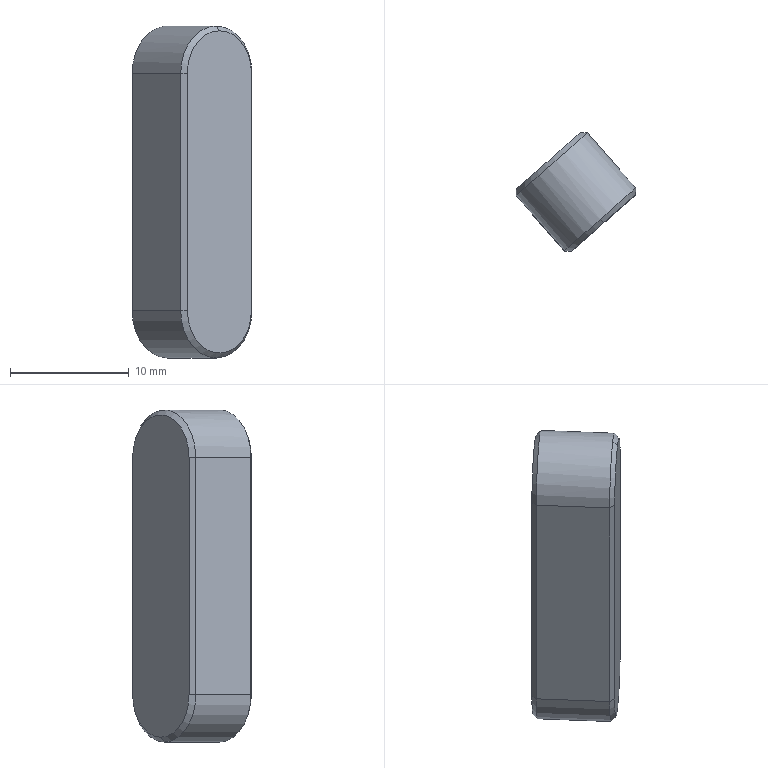Component | SolidWorks | Key8-7-28-1 | 1 solid | 17 faces | box 10.1 x 10.01 x 28 mm | volume 1462 mm3 | plane 8 | cone 6 | cylinder 3 | commonest cylinder face diameters 8 x3
build123d program:
from build123d import *

# Parameters (mm, degrees)
BOSS_EXTRUDE1_DEPTH = 7
CHAMFER1_SIZE2      = 0.4
CHAMFER1_SIZE       = 0.4


with BuildPart() as part:
    # Sketch1 → Boss-Extrude1 (new body)
    with BuildSketch(Plane(origin=(0, 0, 4), x_dir=(1, 0, 0), z_dir=(0, -1, 0))):
        with BuildLine():
            Line((-4, 16), (-4, -4))
            ThreePointArc((-4, -4), (0, -8), (4, -4))
            Line((4, -4), (4, 16))
            ThreePointArc((4, 16), (0, 20), (-4, 16))
        make_face()
    extrude(amount=-BOSS_EXTRUDE1_DEPTH)

    # Chamfer1
    chamfer1_edges = [part.edges().sort_by_distance(p)[0] for p in [
        (0, 7, -4),
        (4, 7, 10),
        (0, 7, 24),
        (4, 0, 10),
        (0, 0, -4),
        (-4, 0, 10),
        (0, 0, 24),
        (-4, 7, 10),
    ]]
    chamfer(chamfer1_edges, length=CHAMFER1_SIZE, length2=CHAMFER1_SIZE2)


solid = part.part

# Placed as in the assembly
solid = solid.moved(Location((-237.022, 13.665, -51.748), (0, 0, -138.66)))
STEP:
#1=CARTESIAN_POINT('',(-9.332,0.538,-2.179));
#2=VERTEX_POINT('',#1);
#3=CARTESIAN_POINT('',(-9.438,0.4444,-2.037));
#4=VERTEX_POINT('',#3);
#5=CARTESIAN_POINT('',(-9.332,0.538,-2.037));
#6=DIRECTION('',(-0.6605,0.7508,-0.));
#7=DIRECTION('',(0.,0.,-1.));
#8=AXIS2_PLACEMENT_3D('',#5,#6,#7);
#9=CIRCLE('',#8,0.1417);
#10=EDGE_CURVE('',#2,#4,#9,.T.);
#11=ORIENTED_EDGE('',*,*,#10,.F.);
#12=CARTESIAN_POINT('',(-9.321,0.5262,-2.195));
#13=VERTEX_POINT('',#12);
#14=CARTESIAN_POINT('',(-9.321,0.5262,-2.195));
#15=DIRECTION('',(0.4671,-0.5309,-0.7071));
#16=VECTOR('',#15,39.37);
#17=LINE('',#14,#16);
#18=EDGE_CURVE('',#2,#13,#17,.T.);
#19=ORIENTED_EDGE('',*,*,#18,.T.);
#20=CARTESIAN_POINT('',(-9.439,0.4221,-2.037));
#21=VERTEX_POINT('',#20);
#22=CARTESIAN_POINT('',(-9.321,0.5262,-2.037));
#23=DIRECTION('',(0.6605,-0.7508,0.));
#24=DIRECTION('',(0.,0.,-1.));
#25=AXIS2_PLACEMENT_3D('',#22,#23,#24);
#26=CIRCLE('',#25,0.1575);
#27=EDGE_CURVE('',#21,#13,#26,.T.);
#28=ORIENTED_EDGE('',*,*,#27,.F.);
#29=CARTESIAN_POINT('',(-9.438,0.4444,-2.037));
#30=DIRECTION('',(-0.06384,-0.998,0.));
#31=VECTOR('',#30,39.37);
#32=LINE('',#29,#31);
#33=EDGE_CURVE('',#4,#21,#32,.T.);
#34=ORIENTED_EDGE('',*,*,#33,.F.);
#35=EDGE_LOOP('',(#11,#19,#28,#34));
#36=FACE_OUTER_BOUND('',#35,.T.);
#37=CARTESIAN_POINT('',(-9.321,0.5262,-2.037));
#38=DIRECTION('',(0.6605,-0.7508,0.));
#39=DIRECTION('',(0.,0.,-1.));
#40=AXIS2_PLACEMENT_3D('',#37,#38,#39);
#41=CONICAL_SURFACE('',#40,0.1575,0.7854);
#42=ADVANCED_FACE('',(#36),#41,.T.);
#43=CARTESIAN_POINT('',(-9.15,0.3311,-1.108));
#44=VERTEX_POINT('',#43);
#45=CARTESIAN_POINT('',(-9.256,0.2374,-1.25));
#46=VERTEX_POINT('',#45);
#47=CARTESIAN_POINT('',(-9.15,0.3311,-1.25));
#48=DIRECTION('',(0.6605,-0.7508,0.));
#49=DIRECTION('',(0.,0.,-1.));
#50=AXIS2_PLACEMENT_3D('',#47,#48,#49);
#51=CIRCLE('',#50,0.1417);
#52=EDGE_CURVE('',#44,#46,#51,.T.);
#53=ORIENTED_EDGE('',*,*,#52,.F.);
#54=CARTESIAN_POINT('',(-9.16,0.3429,-1.092));
#55=VERTEX_POINT('',#54);
#56=CARTESIAN_POINT('',(-9.15,0.3311,-1.108));
#57=DIRECTION('',(-0.4671,0.5309,0.7071));
#58=VECTOR('',#57,39.37);
#59=LINE('',#56,#58);
#60=EDGE_CURVE('',#44,#55,#59,.T.);
#61=ORIENTED_EDGE('',*,*,#60,.T.);
#62=CARTESIAN_POINT('',(-9.278,0.2389,-1.25));
#63=VERTEX_POINT('',#62);
#64=CARTESIAN_POINT('',(-9.16,0.3429,-1.25));
#65=DIRECTION('',(-0.6605,0.7508,-0.));
#66=DIRECTION('',(0.,0.,-1.));
#67=AXIS2_PLACEMENT_3D('',#64,#65,#66);
#68=CIRCLE('',#67,0.1575);
#69=EDGE_CURVE('',#63,#55,#68,.T.);
#70=ORIENTED_EDGE('',*,*,#69,.F.);
#71=CARTESIAN_POINT('',(-9.278,0.2389,-1.25));
#72=DIRECTION('',(0.998,-0.06384,0.));
#73=VECTOR('',#72,39.37);
#74=LINE('',#71,#73);
#75=EDGE_CURVE('',#63,#46,#74,.T.);
#76=ORIENTED_EDGE('',*,*,#75,.T.);
#77=EDGE_LOOP('',(#53,#61,#70,#76));
#78=FACE_OUTER_BOUND('',#77,.T.);
#79=CARTESIAN_POINT('',(-9.15,0.3311,-1.25));
#80=DIRECTION('',(-0.6605,0.7508,-0.));
#81=DIRECTION('',(0.,0.,1.));
#82=AXIS2_PLACEMENT_3D('',#79,#80,#81);
#83=CONICAL_SURFACE('',#82,0.1417,0.7854);
#84=ADVANCED_FACE('',(#78),#83,.T.);
#85=ORIENTED_EDGE('',*,*,#27,.T.);
#86=CARTESIAN_POINT('',(-9.16,0.3429,-2.195));
#87=VERTEX_POINT('',#86);
#88=CARTESIAN_POINT('',(-9.332,0.538,-2.195));
#89=DIRECTION('',(0.6605,-0.7508,0.));
#90=VECTOR('',#89,39.37);
#91=LINE('',#88,#90);
#92=EDGE_CURVE('',#13,#87,#91,.T.);
#93=ORIENTED_EDGE('',*,*,#92,.T.);
#94=CARTESIAN_POINT('',(-9.278,0.2389,-2.037));
#95=VERTEX_POINT('',#94);
#96=CARTESIAN_POINT('',(-9.16,0.3429,-2.037));
#97=DIRECTION('',(-0.6605,0.7508,-0.));
#98=DIRECTION('',(0.,-0.,-1.));
#99=AXIS2_PLACEMENT_3D('',#96,#97,#98);
#100=CIRCLE('',#99,0.1575);
#101=EDGE_CURVE('',#87,#95,#100,.T.);
#102=ORIENTED_EDGE('',*,*,#101,.T.);
#103=CARTESIAN_POINT('',(-9.45,0.434,-2.037));
#104=DIRECTION('',(0.6605,-0.7508,0.));
#105=VECTOR('',#104,39.37);
#106=LINE('',#103,#105);
#107=EDGE_CURVE('',#21,#95,#106,.T.);
#108=ORIENTED_EDGE('',*,*,#107,.F.);
#109=EDGE_LOOP('',(#85,#93,#102,#108));
#110=FACE_OUTER_BOUND('',#109,.T.);
#111=CARTESIAN_POINT('',(-9.332,0.538,-2.037));
#112=DIRECTION('',(0.6605,-0.7508,0.));
#113=DIRECTION('',(0.,0.,-1.));
#114=AXIS2_PLACEMENT_3D('',#111,#112,#113);
#115=CYLINDRICAL_SURFACE('',#114,0.1575);
#116=ADVANCED_FACE('',(#110),#115,.T.);
#117=CARTESIAN_POINT('',(-9.439,0.4221,-1.25));
#118=VERTEX_POINT('',#117);
#119=CARTESIAN_POINT('',(-9.45,0.434,-1.25));
#120=DIRECTION('',(0.6605,-0.7508,0.));
#121=VECTOR('',#120,39.37);
#122=LINE('',#119,#121);
#123=EDGE_CURVE('',#118,#63,#122,.T.);
#124=ORIENTED_EDGE('',*,*,#123,.T.);
#125=ORIENTED_EDGE('',*,*,#69,.T.);
#126=CARTESIAN_POINT('',(-9.042,0.4469,-1.25));
#127=VERTEX_POINT('',#126);
#128=CARTESIAN_POINT('',(-9.16,0.3429,-1.25));
#129=DIRECTION('',(-0.6605,0.7508,-0.));
#130=DIRECTION('',(0.,0.,-1.));
#131=AXIS2_PLACEMENT_3D('',#128,#129,#130);
#132=CIRCLE('',#131,0.1575);
#133=EDGE_CURVE('',#55,#127,#132,.T.);
#134=ORIENTED_EDGE('',*,*,#133,.T.);
#135=CARTESIAN_POINT('',(-9.203,0.6302,-1.25));
#136=VERTEX_POINT('',#135);
#137=CARTESIAN_POINT('',(-9.213,0.642,-1.25));
#138=DIRECTION('',(0.6605,-0.7508,0.));
#139=VECTOR('',#138,39.37);
#140=LINE('',#137,#139);
#141=EDGE_CURVE('',#136,#127,#140,.T.);
#142=ORIENTED_EDGE('',*,*,#141,.F.);
#143=CARTESIAN_POINT('',(-9.321,0.5262,-1.25));
#144=DIRECTION('',(0.6605,-0.7508,0.));
#145=DIRECTION('',(0.,0.,-1.));
#146=AXIS2_PLACEMENT_3D('',#143,#144,#145);
#147=CIRCLE('',#146,0.1575);
#148=EDGE_CURVE('',#136,#118,#147,.T.);
#149=ORIENTED_EDGE('',*,*,#148,.T.);
#150=EDGE_LOOP('',(#124,#125,#134,#142,#149));
#151=FACE_OUTER_BOUND('',#150,.T.);
#152=CARTESIAN_POINT('',(-9.332,0.538,-1.25));
#153=DIRECTION('',(0.6605,-0.7508,0.));
#154=DIRECTION('',(0.,0.,-1.));
#155=AXIS2_PLACEMENT_3D('',#152,#153,#154);
#156=CYLINDRICAL_SURFACE('',#155,0.1575);
#157=ADVANCED_FACE('',(#151),#156,.T.);
#158=ORIENTED_EDGE('',*,*,#141,.T.);
#159=CARTESIAN_POINT('',(-9.042,0.4469,-2.037));
#160=VERTEX_POINT('',#159);
#161=CARTESIAN_POINT('',(-9.042,0.4469,-2.037));
#162=DIRECTION('',(0.,-0.,-1.));
#163=VECTOR('',#162,39.37);
#164=LINE('',#161,#163);
#165=EDGE_CURVE('',#127,#160,#164,.T.);
#166=ORIENTED_EDGE('',*,*,#165,.T.);
#167=CARTESIAN_POINT('',(-9.203,0.6302,-2.037));
#168=VERTEX_POINT('',#167);
#169=CARTESIAN_POINT('',(-9.213,0.642,-2.037));
#170=DIRECTION('',(0.6605,-0.7508,0.));
#171=VECTOR('',#170,39.37);
#172=LINE('',#169,#171);
#173=EDGE_CURVE('',#168,#160,#172,.T.);
#174=ORIENTED_EDGE('',*,*,#173,.F.);
#175=CARTESIAN_POINT('',(-9.203,0.6302,-1.25));
#176=DIRECTION('',(-0.,0.,1.));
#177=VECTOR('',#176,39.37);
#178=LINE('',#175,#177);
#179=EDGE_CURVE('',#168,#136,#178,.T.);
#180=ORIENTED_EDGE('',*,*,#179,.T.);
#181=EDGE_LOOP('',(#158,#166,#174,#180));
#182=FACE_OUTER_BOUND('',#181,.T.);
#183=CARTESIAN_POINT('',(-9.213,0.642,-2.037));
#184=DIRECTION('',(0.7508,0.6605,0.));
#185=DIRECTION('',(0.,-0.,-1.));
#186=AXIS2_PLACEMENT_3D('',#183,#184,#185);
#187=PLANE('',#186);
#188=ADVANCED_FACE('',(#182),#187,.T.);
#189=ORIENTED_EDGE('',*,*,#92,.F.);
#190=CARTESIAN_POINT('',(-9.321,0.5262,-2.037));
#191=DIRECTION('',(0.6605,-0.7508,0.));
#192=DIRECTION('',(0.,0.,-1.));
#193=AXIS2_PLACEMENT_3D('',#190,#191,#192);
#194=CIRCLE('',#193,0.1575);
#195=EDGE_CURVE('',#13,#168,#194,.T.);
#196=ORIENTED_EDGE('',*,*,#195,.T.);
#197=ORIENTED_EDGE('',*,*,#173,.T.);
#198=CARTESIAN_POINT('',(-9.16,0.3429,-2.037));
#199=DIRECTION('',(-0.6605,0.7508,-0.));
#200=DIRECTION('',(0.,0.,-1.));
#201=AXIS2_PLACEMENT_3D('',#198,#199,#200);
#202=CIRCLE('',#201,0.1575);
#203=EDGE_CURVE('',#160,#87,#202,.T.);
#204=ORIENTED_EDGE('',*,*,#203,.T.);
#205=EDGE_LOOP('',(#189,#196,#197,#204));
#206=FACE_OUTER_BOUND('',#205,.T.);
#207=CARTESIAN_POINT('',(-9.332,0.538,-2.037));
#208=DIRECTION('',(0.6605,-0.7508,0.));
#209=DIRECTION('',(0.,0.,-1.));
#210=AXIS2_PLACEMENT_3D('',#207,#208,#209);
#211=CYLINDRICAL_SURFACE('',#210,0.1575);
#212=ADVANCED_FACE('',(#206),#211,.T.);
#213=ORIENTED_EDGE('',*,*,#107,.T.);
#214=CARTESIAN_POINT('',(-9.278,0.2389,-1.25));
#215=DIRECTION('',(-0.,0.,1.));
#216=VECTOR('',#215,39.37);
#217=LINE('',#214,#216);
#218=EDGE_CURVE('',#95,#63,#217,.T.);
#219=ORIENTED_EDGE('',*,*,#218,.T.);
#220=ORIENTED_EDGE('',*,*,#123,.F.);
#221=CARTESIAN_POINT('',(-9.439,0.4221,-2.037));
#222=DIRECTION('',(0.,-0.,-1.));
#223=VECTOR('',#222,39.37);
#224=LINE('',#221,#223);
#225=EDGE_CURVE('',#118,#21,#224,.T.);
#226=ORIENTED_EDGE('',*,*,#225,.T.);
#227=EDGE_LOOP('',(#213,#219,#220,#226));
#228=FACE_OUTER_BOUND('',#227,.T.);
#229=CARTESIAN_POINT('',(-9.45,0.434,-1.25));
#230=DIRECTION('',(-0.7508,-0.6605,-0.));
#231=DIRECTION('',(-0.,0.,1.));
#232=AXIS2_PLACEMENT_3D('',#229,#230,#231);
#233=PLANE('',#232);
#234=ADVANCED_FACE('',(#228),#233,.T.);
#235=CARTESIAN_POINT('',(-9.225,0.6316,-2.037));
#236=VERTEX_POINT('',#235);
#237=CARTESIAN_POINT('',(-9.332,0.538,-2.037));
#238=DIRECTION('',(-0.6605,0.7508,-0.));
#239=DIRECTION('',(0.,-0.,-1.));
#240=AXIS2_PLACEMENT_3D('',#237,#238,#239);
#241=CIRCLE('',#240,0.1417);
#242=EDGE_CURVE('',#236,#2,#241,.T.);
#243=ORIENTED_EDGE('',*,*,#242,.T.);
#244=ORIENTED_EDGE('',*,*,#10,.T.);
#245=CARTESIAN_POINT('',(-9.438,0.4444,-1.25));
#246=VERTEX_POINT('',#245);
#247=CARTESIAN_POINT('',(-9.438,0.4444,-1.25));
#248=DIRECTION('',(-0.,0.,1.));
#249=VECTOR('',#248,39.37);
#250=LINE('',#247,#249);
#251=EDGE_CURVE('',#4,#246,#250,.T.);
#252=ORIENTED_EDGE('',*,*,#251,.T.);
#253=CARTESIAN_POINT('',(-9.225,0.6316,-1.25));
#254=VERTEX_POINT('',#253);
#255=CARTESIAN_POINT('',(-9.332,0.538,-1.25));
#256=DIRECTION('',(-0.6605,0.7508,-0.));
#257=DIRECTION('',(0.,0.,-1.));
#258=AXIS2_PLACEMENT_3D('',#255,#256,#257);
#259=CIRCLE('',#258,0.1417);
#260=EDGE_CURVE('',#246,#254,#259,.T.);
#261=ORIENTED_EDGE('',*,*,#260,.T.);
#262=CARTESIAN_POINT('',(-9.225,0.6316,-2.037));
#263=DIRECTION('',(0.,-0.,-1.));
#264=VECTOR('',#263,39.37);
#265=LINE('',#262,#264);
#266=EDGE_CURVE('',#254,#236,#265,.T.);
#267=ORIENTED_EDGE('',*,*,#266,.T.);
#268=EDGE_LOOP('',(#243,#244,#252,#261,#267));
#269=FACE_OUTER_BOUND('',#268,.T.);
#270=CARTESIAN_POINT('',(-9.332,0.538,-1.25));
#271=DIRECTION('',(0.6605,-0.7508,0.));
#272=DIRECTION('',(0.,-0.,-1.));
#273=AXIS2_PLACEMENT_3D('',#270,#271,#272);
#274=PLANE('',#273);
#275=ADVANCED_FACE('',(#269),#274,.F.);
#276=CARTESIAN_POINT('',(-9.256,0.2374,-2.037));
#277=VERTEX_POINT('',#276);
#278=CARTESIAN_POINT('',(-9.043,0.4247,-2.037));
#279=VERTEX_POINT('',#278);
#280=CARTESIAN_POINT('',(-9.15,0.3311,-2.037));
#281=DIRECTION('',(0.6605,-0.7508,0.));
#282=DIRECTION('',(0.,0.,-1.));
#283=AXIS2_PLACEMENT_3D('',#280,#281,#282);
#284=CIRCLE('',#283,0.1417);
#285=EDGE_CURVE('',#277,#279,#284,.T.);
#286=ORIENTED_EDGE('',*,*,#285,.T.);
#287=CARTESIAN_POINT('',(-9.043,0.4247,-1.25));
#288=VERTEX_POINT('',#287);
#289=CARTESIAN_POINT('',(-9.043,0.4247,-1.25));
#290=DIRECTION('',(-0.,0.,1.));
#291=VECTOR('',#290,39.37);
#292=LINE('',#289,#291);
#293=EDGE_CURVE('',#279,#288,#292,.T.);
#294=ORIENTED_EDGE('',*,*,#293,.T.);
#295=CARTESIAN_POINT('',(-9.15,0.3311,-1.25));
#296=DIRECTION('',(0.6605,-0.7508,0.));
#297=DIRECTION('',(0.,0.,-1.));
#298=AXIS2_PLACEMENT_3D('',#295,#296,#297);
#299=CIRCLE('',#298,0.1417);
#300=EDGE_CURVE('',#288,#44,#299,.T.);
#301=ORIENTED_EDGE('',*,*,#300,.T.);
#302=ORIENTED_EDGE('',*,*,#52,.T.);
#303=CARTESIAN_POINT('',(-9.256,0.2374,-1.25));
#304=DIRECTION('',(0.,-0.,-1.));
#305=VECTOR('',#304,39.37);
#306=LINE('',#303,#305);
#307=EDGE_CURVE('',#46,#277,#306,.T.);
#308=ORIENTED_EDGE('',*,*,#307,.T.);
#309=EDGE_LOOP('',(#286,#294,#301,#302,#308));
#310=FACE_OUTER_BOUND('',#309,.T.);
#311=CARTESIAN_POINT('',(-9.15,0.3311,-1.25));
#312=DIRECTION('',(0.6605,-0.7508,0.));
#313=DIRECTION('',(0.,-0.,-1.));
#314=AXIS2_PLACEMENT_3D('',#311,#312,#313);
#315=PLANE('',#314);
#316=ADVANCED_FACE('',(#310),#315,.T.);
#317=ORIENTED_EDGE('',*,*,#75,.F.);
#318=ORIENTED_EDGE('',*,*,#218,.F.);
#319=CARTESIAN_POINT('',(-9.256,0.2374,-2.037));
#320=DIRECTION('',(-0.998,0.06384,-0.));
#321=VECTOR('',#320,39.37);
#322=LINE('',#319,#321);
#323=EDGE_CURVE('',#277,#95,#322,.T.);
#324=ORIENTED_EDGE('',*,*,#323,.F.);
#325=ORIENTED_EDGE('',*,*,#307,.F.);
#326=EDGE_LOOP('',(#317,#318,#324,#325));
#327=FACE_OUTER_BOUND('',#326,.T.);
#328=CARTESIAN_POINT('',(-9.256,0.2374,-1.25));
#329=DIRECTION('',(0.06384,0.998,-0.));
#330=DIRECTION('',(0.,-0.,-1.));
#331=AXIS2_PLACEMENT_3D('',#328,#329,#330);
#332=PLANE('',#331);
#333=ADVANCED_FACE('',(#327),#332,.F.);
#334=ORIENTED_EDGE('',*,*,#323,.T.);
#335=ORIENTED_EDGE('',*,*,#101,.F.);
#336=ORIENTED_EDGE('',*,*,#203,.F.);
#337=CARTESIAN_POINT('',(-9.043,0.4247,-2.037));
#338=DIRECTION('',(0.06384,0.998,-0.));
#339=VECTOR('',#338,39.37);
#340=LINE('',#337,#339);
#341=EDGE_CURVE('',#279,#160,#340,.T.);
#342=ORIENTED_EDGE('',*,*,#341,.F.);
#343=ORIENTED_EDGE('',*,*,#285,.F.);
#344=EDGE_LOOP('',(#334,#335,#336,#342,#343));
#345=FACE_OUTER_BOUND('',#344,.T.);
#346=CARTESIAN_POINT('',(-9.15,0.3311,-2.037));
#347=DIRECTION('',(-0.6605,0.7508,-0.));
#348=DIRECTION('',(0.,0.,1.));
#349=AXIS2_PLACEMENT_3D('',#346,#347,#348);
#350=CONICAL_SURFACE('',#349,0.1417,0.7854);
#351=ADVANCED_FACE('',(#345),#350,.T.);
#352=ORIENTED_EDGE('',*,*,#60,.F.);
#353=ORIENTED_EDGE('',*,*,#300,.F.);
#354=CARTESIAN_POINT('',(-9.042,0.4469,-1.25));
#355=DIRECTION('',(-0.06384,-0.998,0.));
#356=VECTOR('',#355,39.37);
#357=LINE('',#354,#356);
#358=EDGE_CURVE('',#127,#288,#357,.T.);
#359=ORIENTED_EDGE('',*,*,#358,.F.);
#360=ORIENTED_EDGE('',*,*,#133,.F.);
#361=EDGE_LOOP('',(#352,#353,#359,#360));
#362=FACE_OUTER_BOUND('',#361,.T.);
#363=CARTESIAN_POINT('',(-9.15,0.3311,-1.25));
#364=DIRECTION('',(-0.6605,0.7508,-0.));
#365=DIRECTION('',(0.,0.,1.));
#366=AXIS2_PLACEMENT_3D('',#363,#364,#365);
#367=CONICAL_SURFACE('',#366,0.1417,0.7854);
#368=ADVANCED_FACE('',(#362),#367,.T.);
#369=ORIENTED_EDGE('',*,*,#341,.T.);
#370=ORIENTED_EDGE('',*,*,#165,.F.);
#371=ORIENTED_EDGE('',*,*,#358,.T.);
#372=ORIENTED_EDGE('',*,*,#293,.F.);
#373=EDGE_LOOP('',(#369,#370,#371,#372));
#374=FACE_OUTER_BOUND('',#373,.T.);
#375=CARTESIAN_POINT('',(-9.043,0.4247,-1.25));
#376=DIRECTION('',(-0.998,0.06384,-0.));
#377=DIRECTION('',(-0.,0.,1.));
#378=AXIS2_PLACEMENT_3D('',#375,#376,#377);
#379=PLANE('',#378);
#380=ADVANCED_FACE('',(#374),#379,.F.);
#381=CARTESIAN_POINT('',(-9.225,0.6316,-2.037));
#382=DIRECTION('',(0.998,-0.06384,0.));
#383=VECTOR('',#382,39.37);
#384=LINE('',#381,#383);
#385=EDGE_CURVE('',#236,#168,#384,.T.);
#386=ORIENTED_EDGE('',*,*,#385,.F.);
#387=ORIENTED_EDGE('',*,*,#266,.F.);
#388=CARTESIAN_POINT('',(-9.203,0.6302,-1.25));
#389=DIRECTION('',(-0.998,0.06384,-0.));
#390=VECTOR('',#389,39.37);
#391=LINE('',#388,#390);
#392=EDGE_CURVE('',#136,#254,#391,.T.);
#393=ORIENTED_EDGE('',*,*,#392,.F.);
#394=ORIENTED_EDGE('',*,*,#179,.F.);
#395=EDGE_LOOP('',(#386,#387,#393,#394));
#396=FACE_OUTER_BOUND('',#395,.T.);
#397=CARTESIAN_POINT('',(-9.203,0.6302,-2.037));
#398=DIRECTION('',(0.06384,0.998,-0.));
#399=DIRECTION('',(0.,-0.,-1.));
#400=AXIS2_PLACEMENT_3D('',#397,#398,#399);
#401=PLANE('',#400);
#402=ADVANCED_FACE('',(#396),#401,.T.);
#403=ORIENTED_EDGE('',*,*,#392,.T.);
#404=ORIENTED_EDGE('',*,*,#260,.F.);
#405=CARTESIAN_POINT('',(-9.439,0.4221,-1.25));
#406=DIRECTION('',(0.06384,0.998,-0.));
#407=VECTOR('',#406,39.37);
#408=LINE('',#405,#407);
#409=EDGE_CURVE('',#118,#246,#408,.T.);
#410=ORIENTED_EDGE('',*,*,#409,.F.);
#411=ORIENTED_EDGE('',*,*,#148,.F.);
#412=EDGE_LOOP('',(#403,#404,#410,#411));
#413=FACE_OUTER_BOUND('',#412,.T.);
#414=CARTESIAN_POINT('',(-9.321,0.5262,-1.25));
#415=DIRECTION('',(0.6605,-0.7508,0.));
#416=DIRECTION('',(0.,0.,-1.));
#417=AXIS2_PLACEMENT_3D('',#414,#415,#416);
#418=CONICAL_SURFACE('',#417,0.1575,0.7854);
#419=ADVANCED_FACE('',(#413),#418,.T.);
#420=ORIENTED_EDGE('',*,*,#18,.F.);
#421=ORIENTED_EDGE('',*,*,#242,.F.);
#422=ORIENTED_EDGE('',*,*,#385,.T.);
#423=ORIENTED_EDGE('',*,*,#195,.F.);
#424=EDGE_LOOP('',(#420,#421,#422,#423));
#425=FACE_OUTER_BOUND('',#424,.T.);
#426=CARTESIAN_POINT('',(-9.321,0.5262,-2.037));
#427=DIRECTION('',(0.6605,-0.7508,0.));
#428=DIRECTION('',(0.,0.,-1.));
#429=AXIS2_PLACEMENT_3D('',#426,#427,#428);
#430=CONICAL_SURFACE('',#429,0.1575,0.7854);
#431=ADVANCED_FACE('',(#425),#430,.T.);
#432=ORIENTED_EDGE('',*,*,#409,.T.);
#433=ORIENTED_EDGE('',*,*,#251,.F.);
#434=ORIENTED_EDGE('',*,*,#33,.T.);
#435=ORIENTED_EDGE('',*,*,#225,.F.);
#436=EDGE_LOOP('',(#432,#433,#434,#435));
#437=FACE_OUTER_BOUND('',#436,.T.);
#438=CARTESIAN_POINT('',(-9.439,0.4221,-1.25));
#439=DIRECTION('',(-0.998,0.06384,-0.));
#440=DIRECTION('',(-0.,0.,1.));
#441=AXIS2_PLACEMENT_3D('',#438,#439,#440);
#442=PLANE('',#441);
#443=ADVANCED_FACE('',(#437),#442,.T.);
#444=CLOSED_SHELL('',(#42,#84,#116,#157,#188,#212,#234,#275,#316,#333,#351,#368,#380,#402,#419,#431,#443));
#445=MANIFOLD_SOLID_BREP('',#444);
#446=CARTESIAN_POINT('',(0.,0.,0.));
#447=DIRECTION('',(0.,0.,1.));
#448=DIRECTION('',(1.,0.,0.));
#449=AXIS2_PLACEMENT_3D('',#446,#447,#448);
#450=(LENGTH_UNIT()NAMED_UNIT(*)SI_UNIT($,.METRE.));
#451=LENGTH_MEASURE_WITH_UNIT(LENGTH_MEASURE(0.0254),#450);
#452=DIMENSIONAL_EXPONENTS(1.,0.,0.,0.,0.,0.,0.);
#453=(CONVERSION_BASED_UNIT('',#451)LENGTH_UNIT()NAMED_UNIT(#452));
#454=UNCERTAINTY_MEASURE_WITH_UNIT(LENGTH_MEASURE(0.00001),#453,'','');
#455=(NAMED_UNIT(*)PLANE_ANGLE_UNIT()SI_UNIT($,.RADIAN.));
#456=(NAMED_UNIT(*)SI_UNIT($,.STERADIAN.)SOLID_ANGLE_UNIT());
#457=(GEOMETRIC_REPRESENTATION_CONTEXT(3)GLOBAL_UNCERTAINTY_ASSIGNED_CONTEXT((#454))GLOBAL_UNIT_ASSIGNED_CONTEXT((#453,#455,#456))REPRESENTATION_CONTEXT('',''));
#458=ADVANCED_BREP_SHAPE_REPRESENTATION('',(#445,#449),#457);
#459=COLOUR_RGB('',0.7922,0.8196,0.9333);
#460=FILL_AREA_STYLE_COLOUR('',#459);
#461=FILL_AREA_STYLE('',(#460));
#462=SURFACE_STYLE_FILL_AREA(#461);
#463=SURFACE_SIDE_STYLE('',(#462));
#464=SURFACE_STYLE_USAGE(.BOTH.,#463);
#465=PRESENTATION_STYLE_ASSIGNMENT((#464));
#466=STYLED_ITEM('',(#465),#445);
#467=PRESENTATION_LAYER_ASSIGNMENT('','',(#466));
#468=(LENGTH_UNIT()NAMED_UNIT(*)SI_UNIT($,.METRE.));
#469=LENGTH_MEASURE_WITH_UNIT(LENGTH_MEASURE(0.0254),#468);
#470=DIMENSIONAL_EXPONENTS(1.,0.,0.,0.,0.,0.,0.);
#471=(CONVERSION_BASED_UNIT('',#469)LENGTH_UNIT()NAMED_UNIT(#470));
#472=UNCERTAINTY_MEASURE_WITH_UNIT(LENGTH_MEASURE(0.00001),#471,'','');
#473=(NAMED_UNIT(*)PLANE_ANGLE_UNIT()SI_UNIT($,.RADIAN.));
#474=(NAMED_UNIT(*)SI_UNIT($,.STERADIAN.)SOLID_ANGLE_UNIT());
#475=(GEOMETRIC_REPRESENTATION_CONTEXT(3)GLOBAL_UNCERTAINTY_ASSIGNED_CONTEXT((#472))GLOBAL_UNIT_ASSIGNED_CONTEXT((#471,#473,#474))REPRESENTATION_CONTEXT('',''));
#476=MECHANICAL_DESIGN_GEOMETRIC_PRESENTATION_REPRESENTATION('',(#466),#475);